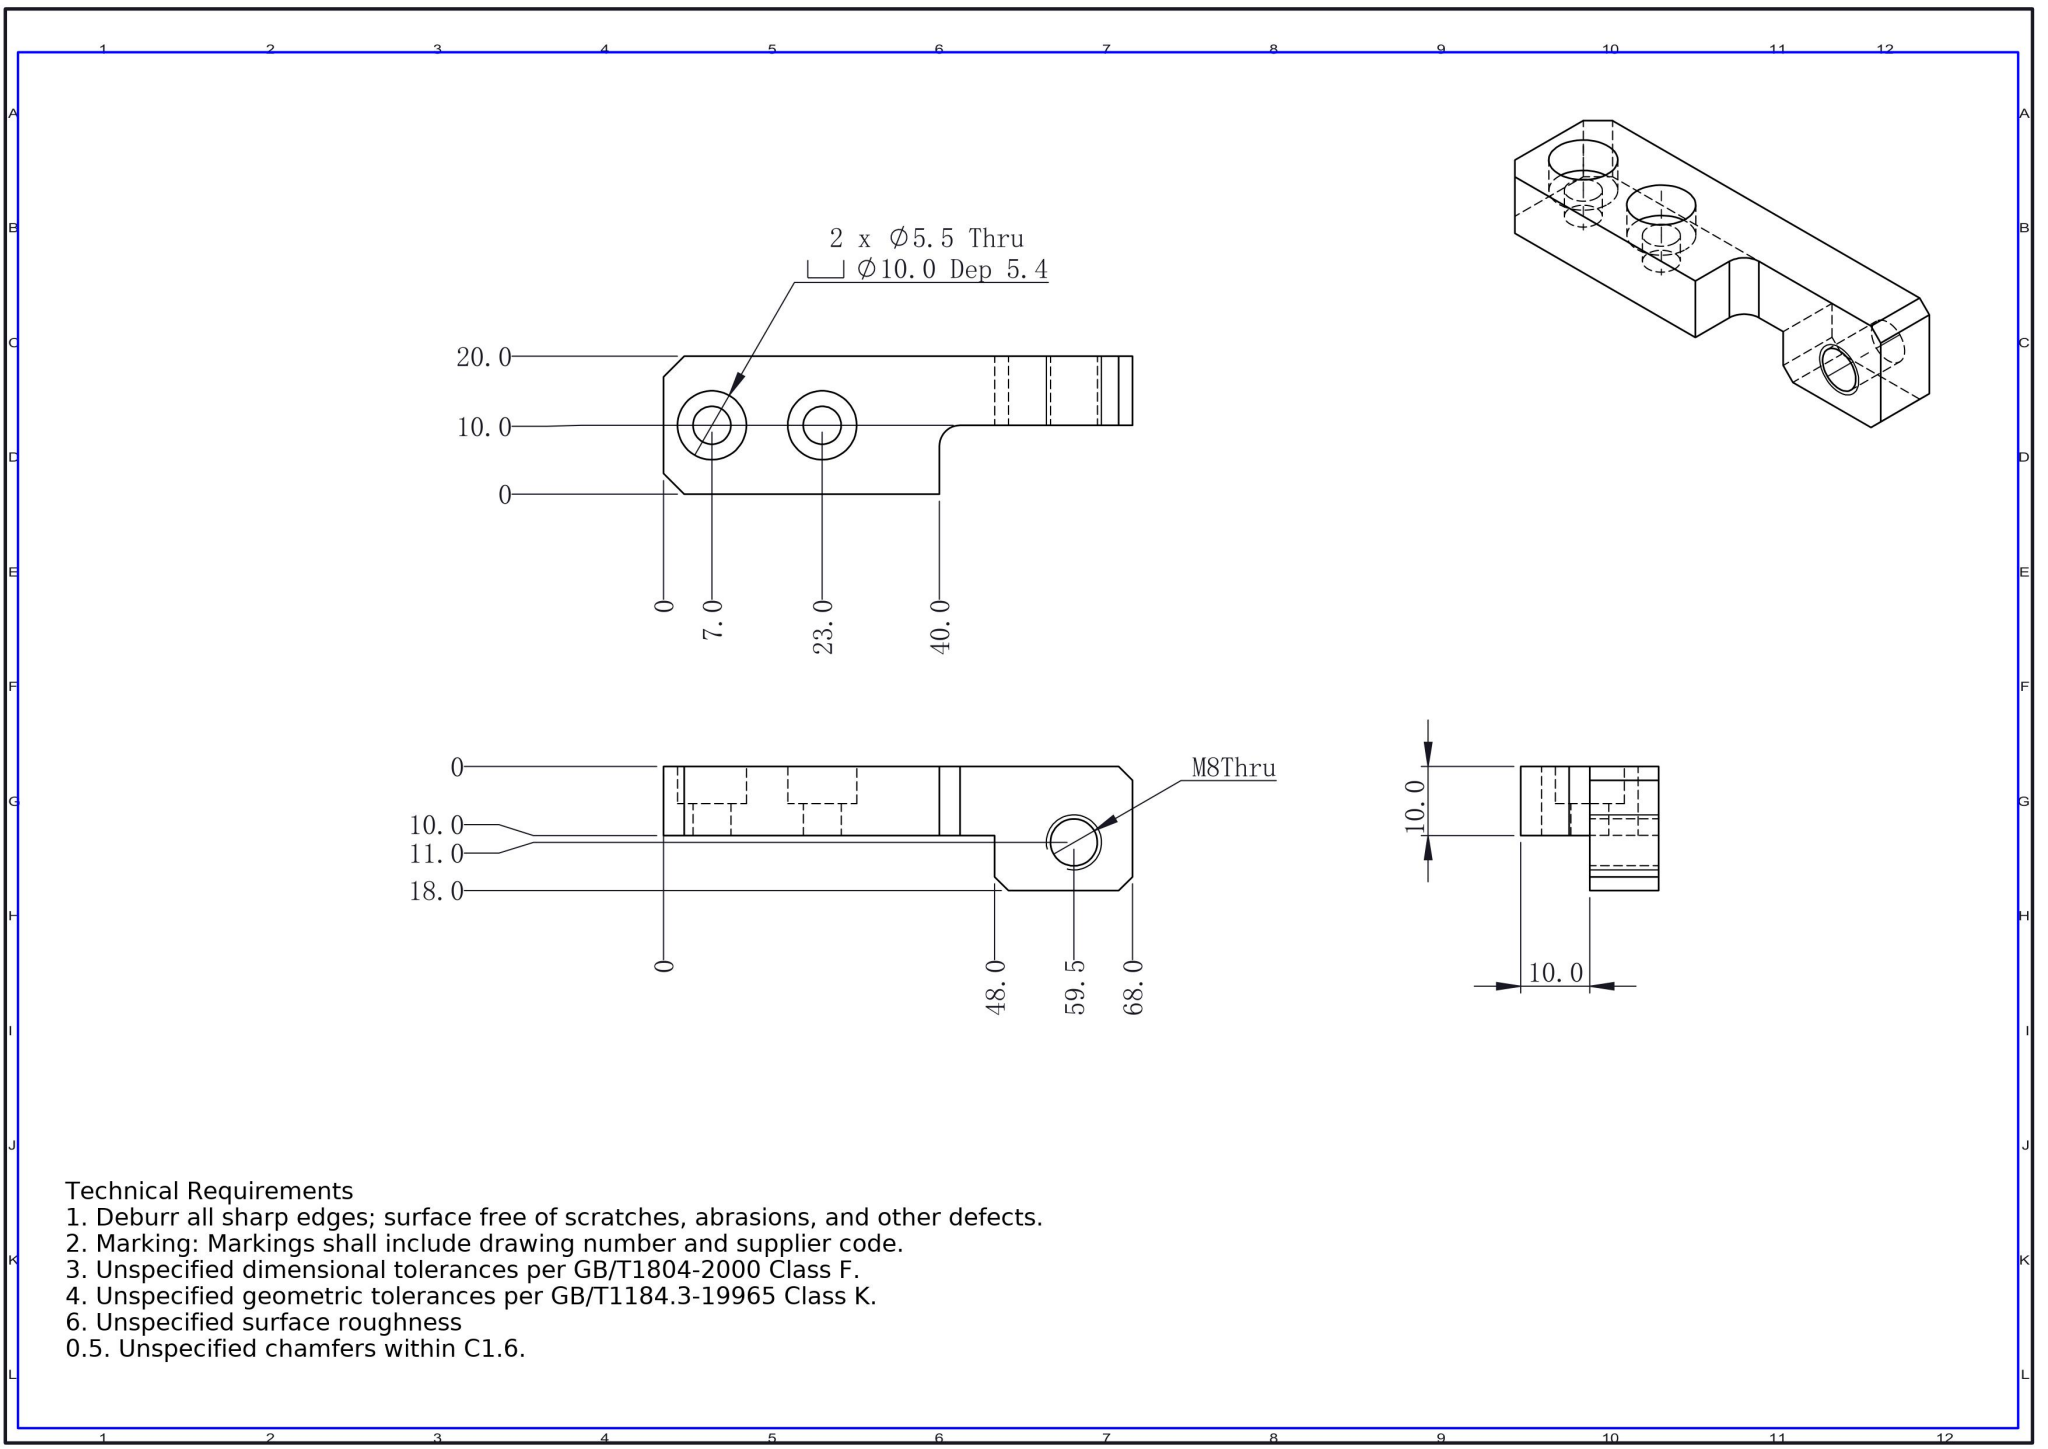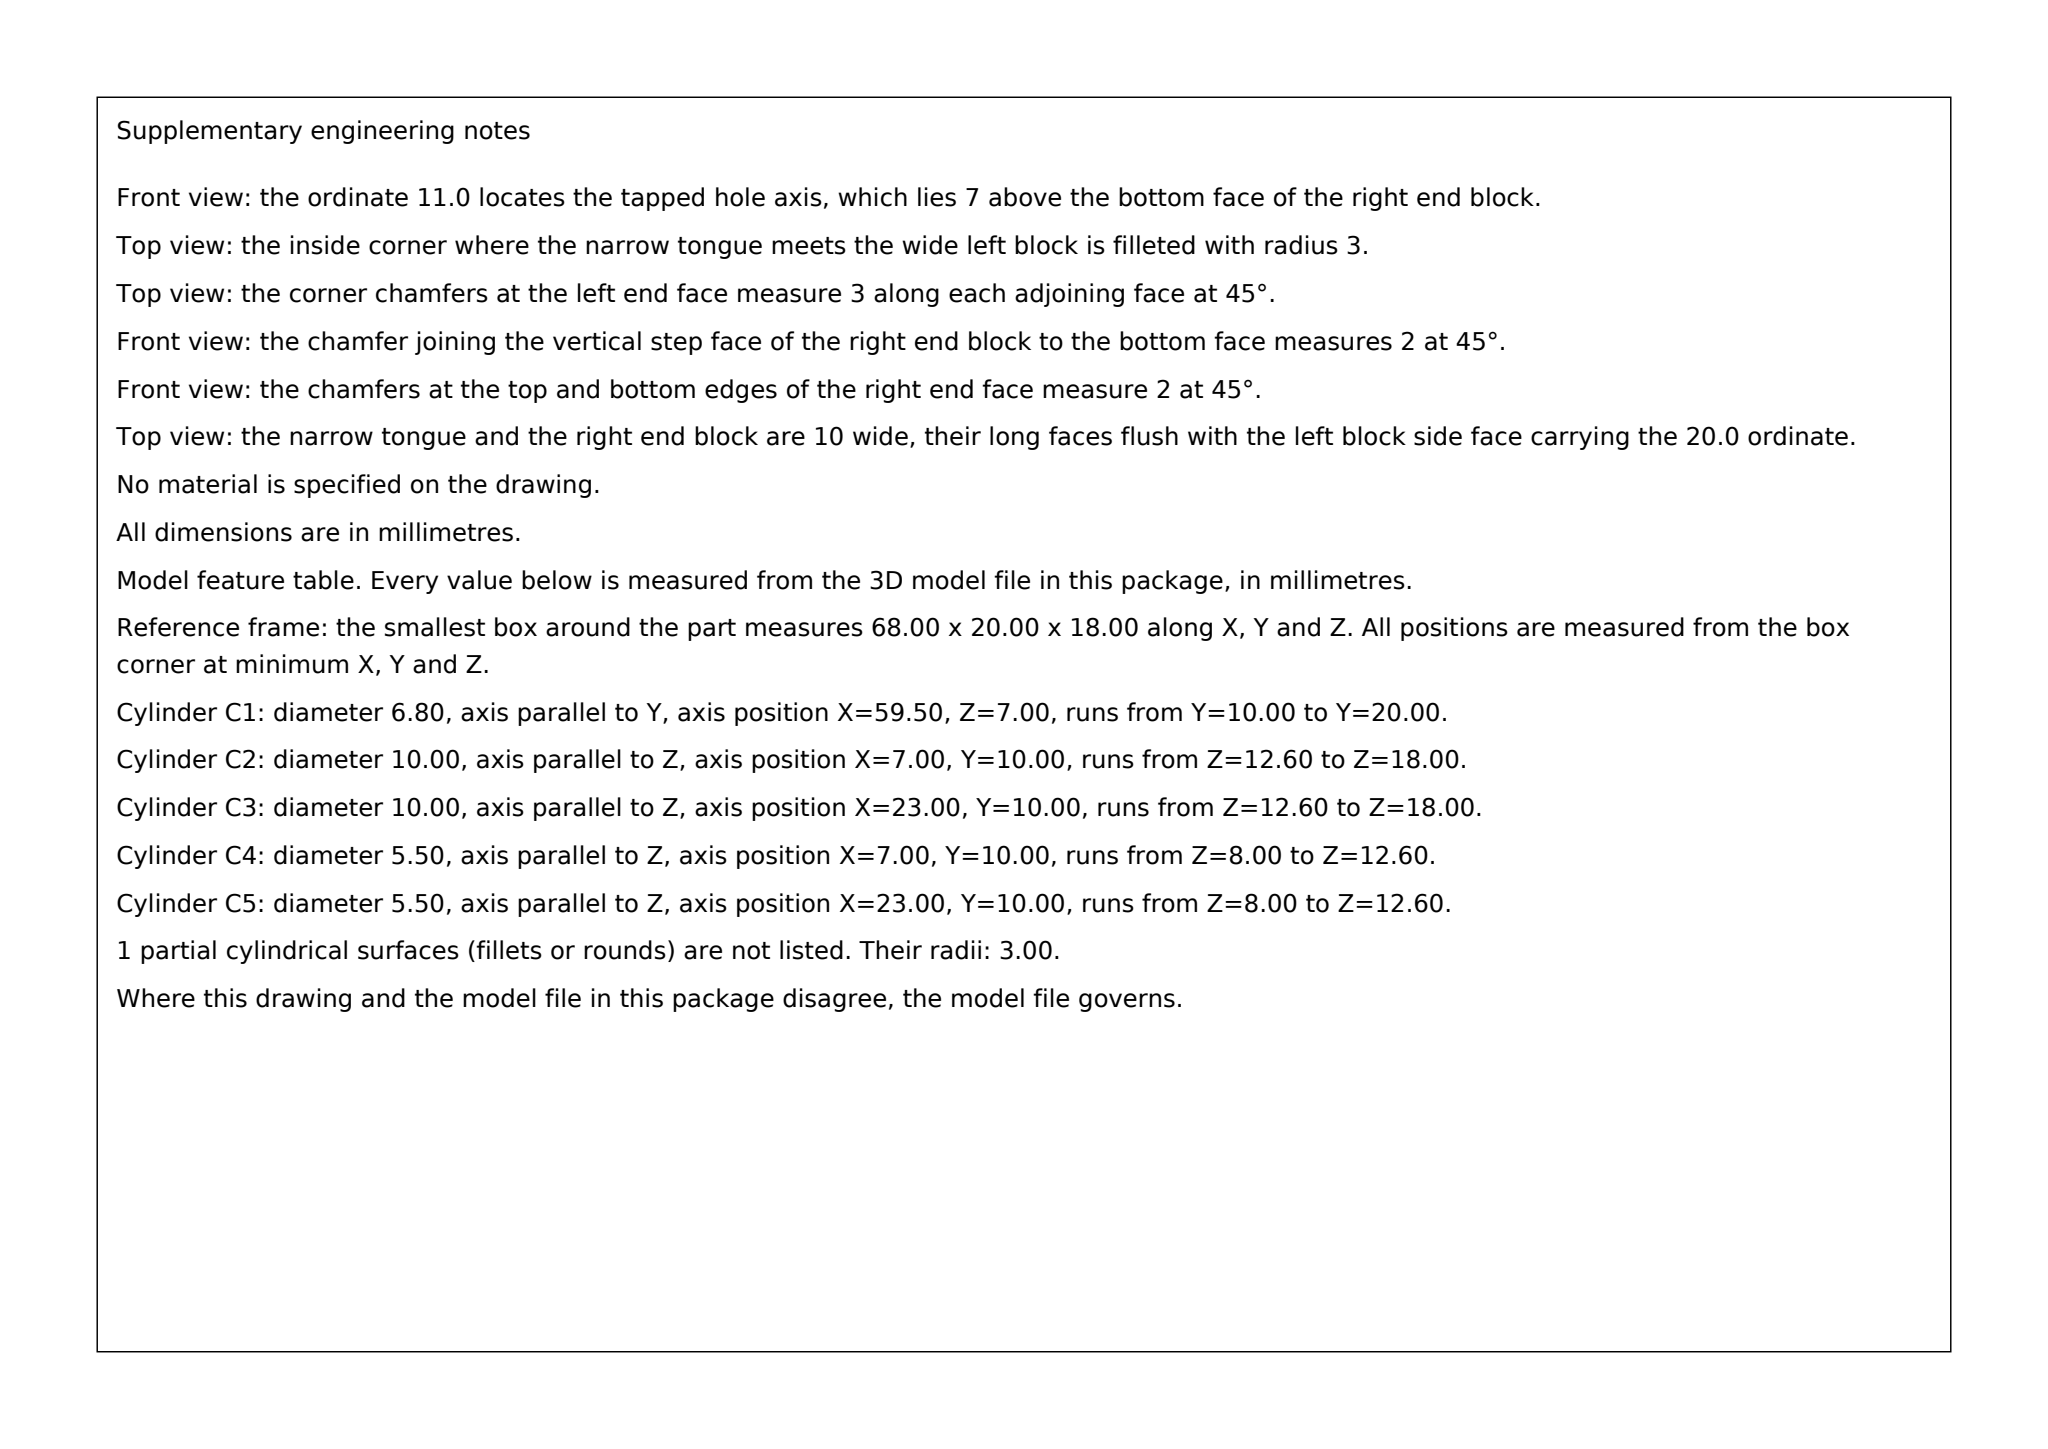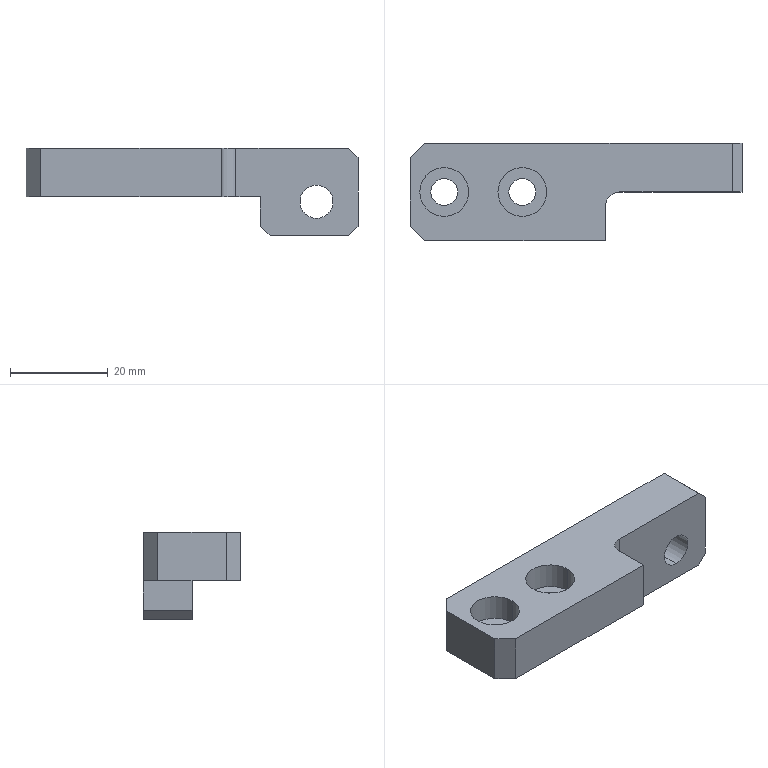Part | SolidWorks | mm | 1 solid | 28 faces | box 68 x 20 x 18 mm | volume 10839 mm3 | plane 17 | cylinder 11 | commonest cylinder face diameters 10 x4 5.5 x4 6.8 x2 6 x1
Drawing notes:
Ø6.0 DP 10.0 FROM TOP FACE; 43.0 FROM LEFT END, 7.0 FROM FRONT EDGE | from the solid: cylinder [6.0,'z',[43.0,7.0,null],10.0]; bbox 68x20x18; z-plane at 8.0 = hole bottom from top face z=18
build123d program:
from build123d import *

# Parameters (mm, degrees)
BOSS_EXTRUDE1_DEPTH                             = 18
M5_HEX_SOCKET_HEAD_CAP_SCREW_CBORE1_D           = 5.5
M5_HEX_SOCKET_HEAD_CAP_SCREW_CBORE1_CBORE_D     = 10
M5_HEX_SOCKET_HEAD_CAP_SCREW_CBORE1_CBORE_DEPTH = 5.4
CHAMFER1_SIZE                                   = 3
FILLET1_R                                       = 3
SKETCH6_W                                       = 48
SKETCH6_H                                       = 8
CUT_EXTRUDE1_DEPTH                              = 74.13
CHAMFER2_SIZE                                   = 2
M8_TAPPED_HOLE1_D                               = 6.8


with BuildPart() as part:
    # Sketch1 → Boss-Extrude1 (new body)
    with BuildSketch(Plane.XY):
        Polygon((0, 0), (68, 0), (68, -10), (40, -10), (40, -20), (0, -20), align=None)
    extrude(amount=BOSS_EXTRUDE1_DEPTH)

    # M5 Hex Socket Head Cap Screw CBORE1 (through all)
    with Locations(Plane.XY.offset(18)):
        with Locations((7, -10), (23, -10)):
            CounterBoreHole(M5_HEX_SOCKET_HEAD_CAP_SCREW_CBORE1_D / 2, M5_HEX_SOCKET_HEAD_CAP_SCREW_CBORE1_CBORE_D / 2, M5_HEX_SOCKET_HEAD_CAP_SCREW_CBORE1_CBORE_DEPTH)

    # Chamfer1
    chamfer1_edges = [part.edges().sort_by_distance(p)[0] for p in [
        (0, 0, 9),
        (0, -20, 9),
    ]]
    chamfer(chamfer1_edges, length=CHAMFER1_SIZE)

    # Fillet1
    fillet1_edges = [part.edges().sort_by_distance(p)[0] for p in [
        (40, -10, 9),
    ]]
    fillet(fillet1_edges, radius=FILLET1_R)

    # Sketch6 → Cut-Extrude1 (cut, through all)
    with BuildSketch(Plane.XZ.offset(20)):
        with Locations((24, 4)):
            Rectangle(SKETCH6_W, SKETCH6_H)
    extrude(amount=-CUT_EXTRUDE1_DEPTH, mode=Mode.SUBTRACT)

    # Chamfer2
    chamfer2_edges = [part.edges().sort_by_distance(p)[0] for p in [
        (68, -5, 18),
        (48, -5, 0),
        (68, -5, 0),
    ]]
    chamfer(chamfer2_edges, length=CHAMFER2_SIZE)

    # M8 Tapped Hole1 (through all)
    with Locations(Plane(origin=(0, -10, 0), x_dir=(-1, 0, 0), z_dir=(0, -1, 0))):
        with Locations((-59.5, -7)):
            Hole(M8_TAPPED_HOLE1_D / 2)


solid = part.part
STEP:
#1=CARTESIAN_POINT('',(59.5,0.,10.4));
#2=VERTEX_POINT('',#1);
#3=CARTESIAN_POINT('',(59.5,0.,3.6));
#4=VERTEX_POINT('',#3);
#5=CARTESIAN_POINT('',(59.5,0.,7.));
#6=DIRECTION('',(0.,-1.,0.));
#7=DIRECTION('',(0.,0.,-1.));
#8=AXIS2_PLACEMENT_3D('',#5,#6,#7);
#9=CIRCLE('',#8,3.4);
#10=EDGE_CURVE('',#2,#4,#9,.T.);
#11=ORIENTED_EDGE('',*,*,#10,.F.);
#12=CARTESIAN_POINT('',(59.5,-10.,10.4));
#13=VERTEX_POINT('',#12);
#14=CARTESIAN_POINT('',(59.5,-10.,10.4));
#15=DIRECTION('',(0.,-1.,0.));
#16=VECTOR('',#15,1000.);
#17=LINE('',#14,#16);
#18=EDGE_CURVE('',#2,#13,#17,.T.);
#19=ORIENTED_EDGE('',*,*,#18,.T.);
#20=CARTESIAN_POINT('',(59.5,-10.,3.6));
#21=VERTEX_POINT('',#20);
#22=CARTESIAN_POINT('',(59.5,-10.,7.));
#23=DIRECTION('',(0.,-1.,0.));
#24=DIRECTION('',(0.,0.,-1.));
#25=AXIS2_PLACEMENT_3D('',#22,#23,#24);
#26=CIRCLE('',#25,3.4);
#27=EDGE_CURVE('',#13,#21,#26,.T.);
#28=ORIENTED_EDGE('',*,*,#27,.T.);
#29=CARTESIAN_POINT('',(59.5,-10.,3.6));
#30=DIRECTION('',(0.,-1.,0.));
#31=VECTOR('',#30,1000.);
#32=LINE('',#29,#31);
#33=EDGE_CURVE('',#4,#21,#32,.T.);
#34=ORIENTED_EDGE('',*,*,#33,.F.);
#35=EDGE_LOOP('',(#11,#19,#28,#34));
#36=FACE_OUTER_BOUND('',#35,.T.);
#37=CARTESIAN_POINT('',(59.5,-10.,7.));
#38=DIRECTION('',(0.,-1.,0.));
#39=DIRECTION('',(0.,0.,-1.));
#40=AXIS2_PLACEMENT_3D('',#37,#38,#39);
#41=CYLINDRICAL_SURFACE('',#40,3.4);
#42=ADVANCED_FACE('',(#36),#41,.F.);
#43=CARTESIAN_POINT('',(2.,-10.,12.6));
#44=VERTEX_POINT('',#43);
#45=CARTESIAN_POINT('',(12.,-10.,12.6));
#46=VERTEX_POINT('',#45);
#47=CARTESIAN_POINT('',(7.,-10.,12.6));
#48=DIRECTION('',(0.,0.,1.));
#49=DIRECTION('',(1.,0.,0.));
#50=AXIS2_PLACEMENT_3D('',#47,#48,#49);
#51=CIRCLE('',#50,5.);
#52=EDGE_CURVE('',#44,#46,#51,.T.);
#53=ORIENTED_EDGE('',*,*,#52,.F.);
#54=CARTESIAN_POINT('',(2.,-10.,18.));
#55=VERTEX_POINT('',#54);
#56=CARTESIAN_POINT('',(2.,-10.,18.));
#57=DIRECTION('',(0.,0.,1.));
#58=VECTOR('',#57,1000.);
#59=LINE('',#56,#58);
#60=EDGE_CURVE('',#44,#55,#59,.T.);
#61=ORIENTED_EDGE('',*,*,#60,.T.);
#62=CARTESIAN_POINT('',(12.,-10.,18.));
#63=VERTEX_POINT('',#62);
#64=CARTESIAN_POINT('',(7.,-10.,18.));
#65=DIRECTION('',(0.,0.,1.));
#66=DIRECTION('',(1.,0.,0.));
#67=AXIS2_PLACEMENT_3D('',#64,#65,#66);
#68=CIRCLE('',#67,5.);
#69=EDGE_CURVE('',#55,#63,#68,.T.);
#70=ORIENTED_EDGE('',*,*,#69,.T.);
#71=CARTESIAN_POINT('',(12.,-10.,18.));
#72=DIRECTION('',(0.,0.,1.));
#73=VECTOR('',#72,1000.);
#74=LINE('',#71,#73);
#75=EDGE_CURVE('',#46,#63,#74,.T.);
#76=ORIENTED_EDGE('',*,*,#75,.F.);
#77=EDGE_LOOP('',(#53,#61,#70,#76));
#78=FACE_OUTER_BOUND('',#77,.T.);
#79=CARTESIAN_POINT('',(7.,-10.,18.));
#80=DIRECTION('',(0.,0.,1.));
#81=DIRECTION('',(1.,0.,0.));
#82=AXIS2_PLACEMENT_3D('',#79,#80,#81);
#83=CYLINDRICAL_SURFACE('',#82,5.);
#84=ADVANCED_FACE('',(#78),#83,.F.);
#85=CARTESIAN_POINT('',(9.75,-10.,8.));
#86=VERTEX_POINT('',#85);
#87=CARTESIAN_POINT('',(4.25,-10.,8.));
#88=VERTEX_POINT('',#87);
#89=CARTESIAN_POINT('',(7.,-10.,8.));
#90=DIRECTION('',(0.,0.,-1.));
#91=DIRECTION('',(1.,0.,0.));
#92=AXIS2_PLACEMENT_3D('',#89,#90,#91);
#93=CIRCLE('',#92,2.75);
#94=EDGE_CURVE('',#86,#88,#93,.T.);
#95=ORIENTED_EDGE('',*,*,#94,.T.);
#96=CARTESIAN_POINT('',(4.25,-10.,12.6));
#97=VERTEX_POINT('',#96);
#98=CARTESIAN_POINT('',(4.25,-10.,18.));
#99=DIRECTION('',(0.,0.,1.));
#100=VECTOR('',#99,1000.);
#101=LINE('',#98,#100);
#102=EDGE_CURVE('',#88,#97,#101,.T.);
#103=ORIENTED_EDGE('',*,*,#102,.T.);
#104=CARTESIAN_POINT('',(9.75,-10.,12.6));
#105=VERTEX_POINT('',#104);
#106=CARTESIAN_POINT('',(7.,-10.,12.6));
#107=DIRECTION('',(0.,0.,1.));
#108=DIRECTION('',(1.,0.,0.));
#109=AXIS2_PLACEMENT_3D('',#106,#107,#108);
#110=CIRCLE('',#109,2.75);
#111=EDGE_CURVE('',#97,#105,#110,.T.);
#112=ORIENTED_EDGE('',*,*,#111,.T.);
#113=CARTESIAN_POINT('',(9.75,-10.,18.));
#114=DIRECTION('',(0.,0.,1.));
#115=VECTOR('',#114,1000.);
#116=LINE('',#113,#115);
#117=EDGE_CURVE('',#86,#105,#116,.T.);
#118=ORIENTED_EDGE('',*,*,#117,.F.);
#119=EDGE_LOOP('',(#95,#103,#112,#118));
#120=FACE_OUTER_BOUND('',#119,.T.);
#121=CARTESIAN_POINT('',(7.,-10.,18.));
#122=DIRECTION('',(0.,0.,1.));
#123=DIRECTION('',(1.,0.,0.));
#124=AXIS2_PLACEMENT_3D('',#121,#122,#123);
#125=CYLINDRICAL_SURFACE('',#124,2.75);
#126=ADVANCED_FACE('',(#120),#125,.F.);
#127=CARTESIAN_POINT('',(18.,-10.,12.6));
#128=VERTEX_POINT('',#127);
#129=CARTESIAN_POINT('',(28.,-10.,12.6));
#130=VERTEX_POINT('',#129);
#131=CARTESIAN_POINT('',(23.,-10.,12.6));
#132=DIRECTION('',(0.,0.,1.));
#133=DIRECTION('',(1.,0.,0.));
#134=AXIS2_PLACEMENT_3D('',#131,#132,#133);
#135=CIRCLE('',#134,5.);
#136=EDGE_CURVE('',#128,#130,#135,.T.);
#137=ORIENTED_EDGE('',*,*,#136,.F.);
#138=CARTESIAN_POINT('',(18.,-10.,18.));
#139=VERTEX_POINT('',#138);
#140=CARTESIAN_POINT('',(18.,-10.,18.));
#141=DIRECTION('',(0.,0.,1.));
#142=VECTOR('',#141,1000.);
#143=LINE('',#140,#142);
#144=EDGE_CURVE('',#128,#139,#143,.T.);
#145=ORIENTED_EDGE('',*,*,#144,.T.);
#146=CARTESIAN_POINT('',(28.,-10.,18.));
#147=VERTEX_POINT('',#146);
#148=CARTESIAN_POINT('',(23.,-10.,18.));
#149=DIRECTION('',(0.,0.,1.));
#150=DIRECTION('',(1.,0.,0.));
#151=AXIS2_PLACEMENT_3D('',#148,#149,#150);
#152=CIRCLE('',#151,5.);
#153=EDGE_CURVE('',#139,#147,#152,.T.);
#154=ORIENTED_EDGE('',*,*,#153,.T.);
#155=CARTESIAN_POINT('',(28.,-10.,18.));
#156=DIRECTION('',(0.,0.,1.));
#157=VECTOR('',#156,1000.);
#158=LINE('',#155,#157);
#159=EDGE_CURVE('',#130,#147,#158,.T.);
#160=ORIENTED_EDGE('',*,*,#159,.F.);
#161=EDGE_LOOP('',(#137,#145,#154,#160));
#162=FACE_OUTER_BOUND('',#161,.T.);
#163=CARTESIAN_POINT('',(23.,-10.,18.));
#164=DIRECTION('',(0.,0.,1.));
#165=DIRECTION('',(1.,0.,0.));
#166=AXIS2_PLACEMENT_3D('',#163,#164,#165);
#167=CYLINDRICAL_SURFACE('',#166,5.);
#168=ADVANCED_FACE('',(#162),#167,.F.);
#169=CARTESIAN_POINT('',(25.75,-10.,8.));
#170=VERTEX_POINT('',#169);
#171=CARTESIAN_POINT('',(20.25,-10.,8.));
#172=VERTEX_POINT('',#171);
#173=CARTESIAN_POINT('',(23.,-10.,8.));
#174=DIRECTION('',(0.,0.,-1.));
#175=DIRECTION('',(1.,0.,0.));
#176=AXIS2_PLACEMENT_3D('',#173,#174,#175);
#177=CIRCLE('',#176,2.75);
#178=EDGE_CURVE('',#170,#172,#177,.T.);
#179=ORIENTED_EDGE('',*,*,#178,.T.);
#180=CARTESIAN_POINT('',(20.25,-10.,12.6));
#181=VERTEX_POINT('',#180);
#182=CARTESIAN_POINT('',(20.25,-10.,18.));
#183=DIRECTION('',(0.,0.,1.));
#184=VECTOR('',#183,1000.);
#185=LINE('',#182,#184);
#186=EDGE_CURVE('',#172,#181,#185,.T.);
#187=ORIENTED_EDGE('',*,*,#186,.T.);
#188=CARTESIAN_POINT('',(25.75,-10.,12.6));
#189=VERTEX_POINT('',#188);
#190=CARTESIAN_POINT('',(23.,-10.,12.6));
#191=DIRECTION('',(0.,0.,1.));
#192=DIRECTION('',(1.,0.,0.));
#193=AXIS2_PLACEMENT_3D('',#190,#191,#192);
#194=CIRCLE('',#193,2.75);
#195=EDGE_CURVE('',#181,#189,#194,.T.);
#196=ORIENTED_EDGE('',*,*,#195,.T.);
#197=CARTESIAN_POINT('',(25.75,-10.,18.));
#198=DIRECTION('',(0.,0.,1.));
#199=VECTOR('',#198,1000.);
#200=LINE('',#197,#199);
#201=EDGE_CURVE('',#170,#189,#200,.T.);
#202=ORIENTED_EDGE('',*,*,#201,.F.);
#203=EDGE_LOOP('',(#179,#187,#196,#202));
#204=FACE_OUTER_BOUND('',#203,.T.);
#205=CARTESIAN_POINT('',(23.,-10.,18.));
#206=DIRECTION('',(0.,0.,1.));
#207=DIRECTION('',(1.,0.,0.));
#208=AXIS2_PLACEMENT_3D('',#205,#206,#207);
#209=CYLINDRICAL_SURFACE('',#208,2.75);
#210=ADVANCED_FACE('',(#204),#209,.F.);
#211=CARTESIAN_POINT('',(0.,-3.,18.));
#212=VERTEX_POINT('',#211);
#213=CARTESIAN_POINT('',(0.,-3.,8.));
#214=VERTEX_POINT('',#213);
#215=CARTESIAN_POINT('',(0.,-3.,18.));
#216=DIRECTION('',(0.,0.,-1.));
#217=VECTOR('',#216,1000.);
#218=LINE('',#215,#217);
#219=EDGE_CURVE('',#212,#214,#218,.T.);
#220=ORIENTED_EDGE('',*,*,#219,.T.);
#221=CARTESIAN_POINT('',(-0.,-17.,8.));
#222=VERTEX_POINT('',#221);
#223=CARTESIAN_POINT('',(0.,0.,8.));
#224=DIRECTION('',(0.,-1.,0.));
#225=VECTOR('',#224,1000.);
#226=LINE('',#223,#225);
#227=EDGE_CURVE('',#214,#222,#226,.T.);
#228=ORIENTED_EDGE('',*,*,#227,.T.);
#229=CARTESIAN_POINT('',(0.,-17.,18.));
#230=VERTEX_POINT('',#229);
#231=CARTESIAN_POINT('',(0.,-17.,18.));
#232=DIRECTION('',(0.,0.,1.));
#233=VECTOR('',#232,1000.);
#234=LINE('',#231,#233);
#235=EDGE_CURVE('',#222,#230,#234,.T.);
#236=ORIENTED_EDGE('',*,*,#235,.T.);
#237=CARTESIAN_POINT('',(0.,0.,18.));
#238=DIRECTION('',(0.,-1.,0.));
#239=VECTOR('',#238,1000.);
#240=LINE('',#237,#239);
#241=EDGE_CURVE('',#212,#230,#240,.T.);
#242=ORIENTED_EDGE('',*,*,#241,.F.);
#243=EDGE_LOOP('',(#220,#228,#236,#242));
#244=FACE_OUTER_BOUND('',#243,.T.);
#245=CARTESIAN_POINT('',(0.,0.,18.));
#246=DIRECTION('',(1.,0.,0.));
#247=DIRECTION('',(0.,0.,-1.));
#248=AXIS2_PLACEMENT_3D('',#245,#246,#247);
#249=PLANE('',#248);
#250=ADVANCED_FACE('',(#244),#249,.F.);
#251=CARTESIAN_POINT('',(3.,-20.,18.));
#252=VERTEX_POINT('',#251);
#253=CARTESIAN_POINT('',(3.,-20.,8.));
#254=VERTEX_POINT('',#253);
#255=CARTESIAN_POINT('',(3.,-20.,18.));
#256=DIRECTION('',(0.,0.,-1.));
#257=VECTOR('',#256,1000.);
#258=LINE('',#255,#257);
#259=EDGE_CURVE('',#252,#254,#258,.T.);
#260=ORIENTED_EDGE('',*,*,#259,.T.);
#261=CARTESIAN_POINT('',(40.,-20.,8.));
#262=VERTEX_POINT('',#261);
#263=CARTESIAN_POINT('',(0.,-20.,8.));
#264=DIRECTION('',(-1.,0.,0.));
#265=VECTOR('',#264,1000.);
#266=LINE('',#263,#265);
#267=EDGE_CURVE('',#262,#254,#266,.T.);
#268=ORIENTED_EDGE('',*,*,#267,.F.);
#269=CARTESIAN_POINT('',(40.,-20.,18.));
#270=VERTEX_POINT('',#269);
#271=CARTESIAN_POINT('',(40.,-20.,18.));
#272=DIRECTION('',(0.,0.,-1.));
#273=VECTOR('',#272,1000.);
#274=LINE('',#271,#273);
#275=EDGE_CURVE('',#270,#262,#274,.T.);
#276=ORIENTED_EDGE('',*,*,#275,.F.);
#277=CARTESIAN_POINT('',(0.,-20.,18.));
#278=DIRECTION('',(1.,0.,0.));
#279=VECTOR('',#278,1000.);
#280=LINE('',#277,#279);
#281=EDGE_CURVE('',#252,#270,#280,.T.);
#282=ORIENTED_EDGE('',*,*,#281,.F.);
#283=EDGE_LOOP('',(#260,#268,#276,#282));
#284=FACE_OUTER_BOUND('',#283,.T.);
#285=CARTESIAN_POINT('',(0.,-20.,18.));
#286=DIRECTION('',(0.,1.,0.));
#287=DIRECTION('',(0.,0.,1.));
#288=AXIS2_PLACEMENT_3D('',#285,#286,#287);
#289=PLANE('',#288);
#290=ADVANCED_FACE('',(#284),#289,.F.);
#291=ORIENTED_EDGE('',*,*,#275,.T.);
#292=CARTESIAN_POINT('',(40.,-13.,8.));
#293=VERTEX_POINT('',#292);
#294=CARTESIAN_POINT('',(40.,-20.,8.));
#295=DIRECTION('',(0.,1.,0.));
#296=VECTOR('',#295,1000.);
#297=LINE('',#294,#296);
#298=EDGE_CURVE('',#262,#293,#297,.T.);
#299=ORIENTED_EDGE('',*,*,#298,.T.);
#300=CARTESIAN_POINT('',(40.,-13.,18.));
#301=VERTEX_POINT('',#300);
#302=CARTESIAN_POINT('',(40.,-13.,18.));
#303=DIRECTION('',(0.,0.,1.));
#304=VECTOR('',#303,1000.);
#305=LINE('',#302,#304);
#306=EDGE_CURVE('',#293,#301,#305,.T.);
#307=ORIENTED_EDGE('',*,*,#306,.T.);
#308=CARTESIAN_POINT('',(40.,-20.,18.));
#309=DIRECTION('',(0.,1.,0.));
#310=VECTOR('',#309,1000.);
#311=LINE('',#308,#310);
#312=EDGE_CURVE('',#270,#301,#311,.T.);
#313=ORIENTED_EDGE('',*,*,#312,.F.);
#314=EDGE_LOOP('',(#291,#299,#307,#313));
#315=FACE_OUTER_BOUND('',#314,.T.);
#316=CARTESIAN_POINT('',(40.,-20.,18.));
#317=DIRECTION('',(-1.,0.,0.));
#318=DIRECTION('',(0.,0.,1.));
#319=AXIS2_PLACEMENT_3D('',#316,#317,#318);
#320=PLANE('',#319);
#321=ADVANCED_FACE('',(#315),#320,.F.);
#322=CARTESIAN_POINT('',(59.5,-10.,7.));
#323=DIRECTION('',(0.,-1.,0.));
#324=DIRECTION('',(0.,0.,-1.));
#325=AXIS2_PLACEMENT_3D('',#322,#323,#324);
#326=CIRCLE('',#325,3.4);
#327=EDGE_CURVE('',#21,#13,#326,.T.);
#328=ORIENTED_EDGE('',*,*,#327,.F.);
#329=ORIENTED_EDGE('',*,*,#27,.F.);
#330=EDGE_LOOP('',(#328,#329));
#331=FACE_BOUND('',#330,.T.);
#332=CARTESIAN_POINT('',(48.,-10.,8.));
#333=VERTEX_POINT('',#332);
#334=CARTESIAN_POINT('',(48.,-10.,2.));
#335=VERTEX_POINT('',#334);
#336=CARTESIAN_POINT('',(48.,-10.,18.));
#337=DIRECTION('',(0.,0.,-1.));
#338=VECTOR('',#337,1000.);
#339=LINE('',#336,#338);
#340=EDGE_CURVE('',#333,#335,#339,.T.);
#341=ORIENTED_EDGE('',*,*,#340,.T.);
#342=CARTESIAN_POINT('',(50.,-10.,0.));
#343=VERTEX_POINT('',#342);
#344=CARTESIAN_POINT('',(48.,-10.,2.));
#345=DIRECTION('',(0.7071,0.,-0.7071));
#346=VECTOR('',#345,1000.);
#347=LINE('',#344,#346);
#348=EDGE_CURVE('',#335,#343,#347,.T.);
#349=ORIENTED_EDGE('',*,*,#348,.T.);
#350=CARTESIAN_POINT('',(66.,-10.,0.));
#351=VERTEX_POINT('',#350);
#352=CARTESIAN_POINT('',(68.,-10.,0.));
#353=DIRECTION('',(1.,0.,0.));
#354=VECTOR('',#353,1000.);
#355=LINE('',#352,#354);
#356=EDGE_CURVE('',#343,#351,#355,.T.);
#357=ORIENTED_EDGE('',*,*,#356,.T.);
#358=CARTESIAN_POINT('',(68.,-10.,2.));
#359=VERTEX_POINT('',#358);
#360=CARTESIAN_POINT('',(68.,-10.,2.));
#361=DIRECTION('',(0.7071,0.,0.7071));
#362=VECTOR('',#361,1000.);
#363=LINE('',#360,#362);
#364=EDGE_CURVE('',#351,#359,#363,.T.);
#365=ORIENTED_EDGE('',*,*,#364,.T.);
#366=CARTESIAN_POINT('',(68.,-10.,16.));
#367=VERTEX_POINT('',#366);
#368=CARTESIAN_POINT('',(68.,-10.,18.));
#369=DIRECTION('',(0.,0.,-1.));
#370=VECTOR('',#369,1000.);
#371=LINE('',#368,#370);
#372=EDGE_CURVE('',#367,#359,#371,.T.);
#373=ORIENTED_EDGE('',*,*,#372,.F.);
#374=CARTESIAN_POINT('',(66.,-10.,18.));
#375=VERTEX_POINT('',#374);
#376=CARTESIAN_POINT('',(66.,-10.,18.));
#377=DIRECTION('',(-0.7071,-0.,0.7071));
#378=VECTOR('',#377,1000.);
#379=LINE('',#376,#378);
#380=EDGE_CURVE('',#367,#375,#379,.T.);
#381=ORIENTED_EDGE('',*,*,#380,.T.);
#382=CARTESIAN_POINT('',(43.,-10.,18.));
#383=VERTEX_POINT('',#382);
#384=CARTESIAN_POINT('',(68.,-10.,18.));
#385=DIRECTION('',(1.,0.,0.));
#386=VECTOR('',#385,1000.);
#387=LINE('',#384,#386);
#388=EDGE_CURVE('',#383,#375,#387,.T.);
#389=ORIENTED_EDGE('',*,*,#388,.F.);
#390=CARTESIAN_POINT('',(43.,-10.,8.));
#391=VERTEX_POINT('',#390);
#392=CARTESIAN_POINT('',(43.,-10.,0.));
#393=DIRECTION('',(0.,0.,-1.));
#394=VECTOR('',#393,1000.);
#395=LINE('',#392,#394);
#396=EDGE_CURVE('',#383,#391,#395,.T.);
#397=ORIENTED_EDGE('',*,*,#396,.T.);
#398=CARTESIAN_POINT('',(68.,-10.,8.));
#399=DIRECTION('',(1.,0.,0.));
#400=VECTOR('',#399,1000.);
#401=LINE('',#398,#400);
#402=EDGE_CURVE('',#391,#333,#401,.T.);
#403=ORIENTED_EDGE('',*,*,#402,.T.);
#404=EDGE_LOOP('',(#341,#349,#357,#365,#373,#381,#389,#397,#403));
#405=FACE_OUTER_BOUND('',#404,.T.);
#406=CARTESIAN_POINT('',(68.,-10.,18.));
#407=DIRECTION('',(-0.,1.,0.));
#408=DIRECTION('',(-1.,-0.,0.));
#409=AXIS2_PLACEMENT_3D('',#406,#407,#408);
#410=PLANE('',#409);
#411=ADVANCED_FACE('',(#331,#405),#410,.F.);
#412=ORIENTED_EDGE('',*,*,#372,.T.);
#413=CARTESIAN_POINT('',(68.,0.,2.));
#414=VERTEX_POINT('',#413);
#415=CARTESIAN_POINT('',(68.,0.,2.));
#416=DIRECTION('',(0.,1.,0.));
#417=VECTOR('',#416,1000.);
#418=LINE('',#415,#417);
#419=EDGE_CURVE('',#359,#414,#418,.T.);
#420=ORIENTED_EDGE('',*,*,#419,.T.);
#421=CARTESIAN_POINT('',(68.,0.,16.));
#422=VERTEX_POINT('',#421);
#423=CARTESIAN_POINT('',(68.,0.,18.));
#424=DIRECTION('',(0.,0.,-1.));
#425=VECTOR('',#424,1000.);
#426=LINE('',#423,#425);
#427=EDGE_CURVE('',#422,#414,#426,.T.);
#428=ORIENTED_EDGE('',*,*,#427,.F.);
#429=CARTESIAN_POINT('',(68.,-10.,16.));
#430=DIRECTION('',(0.,-1.,0.));
#431=VECTOR('',#430,1000.);
#432=LINE('',#429,#431);
#433=EDGE_CURVE('',#422,#367,#432,.T.);
#434=ORIENTED_EDGE('',*,*,#433,.T.);
#435=EDGE_LOOP('',(#412,#420,#428,#434));
#436=FACE_OUTER_BOUND('',#435,.T.);
#437=CARTESIAN_POINT('',(68.,0.,18.));
#438=DIRECTION('',(-1.,0.,0.));
#439=DIRECTION('',(0.,0.,1.));
#440=AXIS2_PLACEMENT_3D('',#437,#438,#439);
#441=PLANE('',#440);
#442=ADVANCED_FACE('',(#436),#441,.F.);
#443=CARTESIAN_POINT('',(59.5,0.,7.));
#444=DIRECTION('',(0.,-1.,0.));
#445=DIRECTION('',(0.,0.,-1.));
#446=AXIS2_PLACEMENT_3D('',#443,#444,#445);
#447=CIRCLE('',#446,3.4);
#448=EDGE_CURVE('',#4,#2,#447,.T.);
#449=ORIENTED_EDGE('',*,*,#448,.T.);
#450=ORIENTED_EDGE('',*,*,#10,.T.);
#451=EDGE_LOOP('',(#449,#450));
#452=FACE_BOUND('',#451,.T.);
#453=CARTESIAN_POINT('',(66.,0.,0.));
#454=VERTEX_POINT('',#453);
#455=CARTESIAN_POINT('',(50.,0.,0.));
#456=VERTEX_POINT('',#455);
#457=CARTESIAN_POINT('',(0.,0.,0.));
#458=DIRECTION('',(-1.,0.,0.));
#459=VECTOR('',#458,1000.);
#460=LINE('',#457,#459);
#461=EDGE_CURVE('',#454,#456,#460,.T.);
#462=ORIENTED_EDGE('',*,*,#461,.T.);
#463=CARTESIAN_POINT('',(48.,0.,2.));
#464=VERTEX_POINT('',#463);
#465=CARTESIAN_POINT('',(48.,0.,2.));
#466=DIRECTION('',(-0.7071,0.,0.7071));
#467=VECTOR('',#466,1000.);
#468=LINE('',#465,#467);
#469=EDGE_CURVE('',#456,#464,#468,.T.);
#470=ORIENTED_EDGE('',*,*,#469,.T.);
#471=CARTESIAN_POINT('',(48.,0.,8.));
#472=VERTEX_POINT('',#471);
#473=CARTESIAN_POINT('',(48.,0.,0.));
#474=DIRECTION('',(0.,0.,1.));
#475=VECTOR('',#474,1000.);
#476=LINE('',#473,#475);
#477=EDGE_CURVE('',#464,#472,#476,.T.);
#478=ORIENTED_EDGE('',*,*,#477,.T.);
#479=CARTESIAN_POINT('',(3.,0.,8.));
#480=VERTEX_POINT('',#479);
#481=CARTESIAN_POINT('',(0.,0.,8.));
#482=DIRECTION('',(-1.,0.,0.));
#483=VECTOR('',#482,1000.);
#484=LINE('',#481,#483);
#485=EDGE_CURVE('',#472,#480,#484,.T.);
#486=ORIENTED_EDGE('',*,*,#485,.T.);
#487=CARTESIAN_POINT('',(3.,0.,18.));
#488=VERTEX_POINT('',#487);
#489=CARTESIAN_POINT('',(3.,0.,18.));
#490=DIRECTION('',(0.,0.,1.));
#491=VECTOR('',#490,1000.);
#492=LINE('',#489,#491);
#493=EDGE_CURVE('',#480,#488,#492,.T.);
#494=ORIENTED_EDGE('',*,*,#493,.T.);
#495=CARTESIAN_POINT('',(66.,0.,18.));
#496=VERTEX_POINT('',#495);
#497=CARTESIAN_POINT('',(0.,0.,18.));
#498=DIRECTION('',(-1.,0.,0.));
#499=VECTOR('',#498,1000.);
#500=LINE('',#497,#499);
#501=EDGE_CURVE('',#496,#488,#500,.T.);
#502=ORIENTED_EDGE('',*,*,#501,.F.);
#503=CARTESIAN_POINT('',(66.,0.,18.));
#504=DIRECTION('',(0.7071,0.,-0.7071));
#505=VECTOR('',#504,1000.);
#506=LINE('',#503,#505);
#507=EDGE_CURVE('',#496,#422,#506,.T.);
#508=ORIENTED_EDGE('',*,*,#507,.T.);
#509=ORIENTED_EDGE('',*,*,#427,.T.);
#510=CARTESIAN_POINT('',(68.,0.,2.));
#511=DIRECTION('',(-0.7071,0.,-0.7071));
#512=VECTOR('',#511,1000.);
#513=LINE('',#510,#512);
#514=EDGE_CURVE('',#414,#454,#513,.T.);
#515=ORIENTED_EDGE('',*,*,#514,.T.);
#516=EDGE_LOOP('',(#462,#470,#478,#486,#494,#502,#508,#509,#515));
#517=FACE_OUTER_BOUND('',#516,.T.);
#518=CARTESIAN_POINT('',(0.,0.,18.));
#519=DIRECTION('',(0.,-1.,0.));
#520=DIRECTION('',(0.,0.,-1.));
#521=AXIS2_PLACEMENT_3D('',#518,#519,#520);
#522=PLANE('',#521);
#523=ADVANCED_FACE('',(#452,#517),#522,.F.);
#524=CARTESIAN_POINT('',(7.,-10.,18.));
#525=DIRECTION('',(0.,0.,1.));
#526=DIRECTION('',(1.,0.,0.));
#527=AXIS2_PLACEMENT_3D('',#524,#525,#526);
#528=CIRCLE('',#527,5.);
#529=EDGE_CURVE('',#63,#55,#528,.T.);
#530=ORIENTED_EDGE('',*,*,#529,.F.);
#531=ORIENTED_EDGE('',*,*,#69,.F.);
#532=EDGE_LOOP('',(#530,#531));
#533=FACE_BOUND('',#532,.T.);
#534=CARTESIAN_POINT('',(23.,-10.,18.));
#535=DIRECTION('',(0.,0.,1.));
#536=DIRECTION('',(1.,0.,0.));
#537=AXIS2_PLACEMENT_3D('',#534,#535,#536);
#538=CIRCLE('',#537,5.);
#539=EDGE_CURVE('',#147,#139,#538,.T.);
#540=ORIENTED_EDGE('',*,*,#539,.F.);
#541=ORIENTED_EDGE('',*,*,#153,.F.);
#542=EDGE_LOOP('',(#540,#541));
#543=FACE_BOUND('',#542,.T.);
#544=ORIENTED_EDGE('',*,*,#388,.T.);
#545=CARTESIAN_POINT('',(66.,0.,18.));
#546=DIRECTION('',(0.,1.,0.));
#547=VECTOR('',#546,1000.);
#548=LINE('',#545,#547);
#549=EDGE_CURVE('',#375,#496,#548,.T.);
#550=ORIENTED_EDGE('',*,*,#549,.T.);
#551=ORIENTED_EDGE('',*,*,#501,.T.);
#552=CARTESIAN_POINT('',(1.5,-1.5,18.));
#553=DIRECTION('',(-0.7071,-0.7071,0.));
#554=VECTOR('',#553,1000.);
#555=LINE('',#552,#554);
#556=EDGE_CURVE('',#488,#212,#555,.T.);
#557=ORIENTED_EDGE('',*,*,#556,.T.);
#558=ORIENTED_EDGE('',*,*,#241,.T.);
#559=CARTESIAN_POINT('',(-8.5,-8.5,18.));
#560=DIRECTION('',(0.7071,-0.7071,0.));
#561=VECTOR('',#560,1000.);
#562=LINE('',#559,#561);
#563=EDGE_CURVE('',#230,#252,#562,.T.);
#564=ORIENTED_EDGE('',*,*,#563,.T.);
#565=ORIENTED_EDGE('',*,*,#281,.T.);
#566=ORIENTED_EDGE('',*,*,#312,.T.);
#567=CARTESIAN_POINT('',(43.,-13.,18.));
#568=DIRECTION('',(0.,0.,-1.));
#569=DIRECTION('',(1.,0.,0.));
#570=AXIS2_PLACEMENT_3D('',#567,#568,#569);
#571=CIRCLE('',#570,3.);
#572=EDGE_CURVE('',#301,#383,#571,.T.);
#573=ORIENTED_EDGE('',*,*,#572,.T.);
#574=EDGE_LOOP('',(#544,#550,#551,#557,#558,#564,#565,#566,#573));
#575=FACE_OUTER_BOUND('',#574,.T.);
#576=CARTESIAN_POINT('',(0.,0.,18.));
#577=DIRECTION('',(0.,0.,1.));
#578=DIRECTION('',(1.,0.,0.));
#579=AXIS2_PLACEMENT_3D('',#576,#577,#578);
#580=PLANE('',#579);
#581=ADVANCED_FACE('',(#533,#543,#575),#580,.T.);
#582=ORIENTED_EDGE('',*,*,#356,.F.);
#583=CARTESIAN_POINT('',(50.,0.,0.));
#584=DIRECTION('',(0.,1.,0.));
#585=VECTOR('',#584,1000.);
#586=LINE('',#583,#585);
#587=EDGE_CURVE('',#343,#456,#586,.T.);
#588=ORIENTED_EDGE('',*,*,#587,.T.);
#589=ORIENTED_EDGE('',*,*,#461,.F.);
#590=CARTESIAN_POINT('',(66.,0.,0.));
#591=DIRECTION('',(0.,-1.,0.));
#592=VECTOR('',#591,1000.);
#593=LINE('',#590,#592);
#594=EDGE_CURVE('',#454,#351,#593,.T.);
#595=ORIENTED_EDGE('',*,*,#594,.T.);
#596=EDGE_LOOP('',(#582,#588,#589,#595));
#597=FACE_OUTER_BOUND('',#596,.T.);
#598=CARTESIAN_POINT('',(0.,0.,0.));
#599=DIRECTION('',(0.,0.,1.));
#600=DIRECTION('',(1.,0.,0.));
#601=AXIS2_PLACEMENT_3D('',#598,#599,#600);
#602=PLANE('',#601);
#603=ADVANCED_FACE('',(#597),#602,.F.);
#604=ORIENTED_EDGE('',*,*,#186,.F.);
#605=CARTESIAN_POINT('',(23.,-10.,8.));
#606=DIRECTION('',(0.,0.,-1.));
#607=DIRECTION('',(1.,0.,0.));
#608=AXIS2_PLACEMENT_3D('',#605,#606,#607);
#609=CIRCLE('',#608,2.75);
#610=EDGE_CURVE('',#172,#170,#609,.T.);
#611=ORIENTED_EDGE('',*,*,#610,.T.);
#612=ORIENTED_EDGE('',*,*,#201,.T.);
#613=CARTESIAN_POINT('',(23.,-10.,12.6));
#614=DIRECTION('',(0.,0.,1.));
#615=DIRECTION('',(1.,0.,0.));
#616=AXIS2_PLACEMENT_3D('',#613,#614,#615);
#617=CIRCLE('',#616,2.75);
#618=EDGE_CURVE('',#189,#181,#617,.T.);
#619=ORIENTED_EDGE('',*,*,#618,.T.);
#620=EDGE_LOOP('',(#604,#611,#612,#619));
#621=FACE_OUTER_BOUND('',#620,.T.);
#622=CARTESIAN_POINT('',(23.,-10.,18.));
#623=DIRECTION('',(0.,0.,1.));
#624=DIRECTION('',(1.,0.,0.));
#625=AXIS2_PLACEMENT_3D('',#622,#623,#624);
#626=CYLINDRICAL_SURFACE('',#625,2.75);
#627=ADVANCED_FACE('',(#621),#626,.F.);
#628=ORIENTED_EDGE('',*,*,#618,.F.);
#629=ORIENTED_EDGE('',*,*,#195,.F.);
#630=EDGE_LOOP('',(#628,#629));
#631=FACE_BOUND('',#630,.T.);
#632=CARTESIAN_POINT('',(23.,-10.,12.6));
#633=DIRECTION('',(0.,0.,1.));
#634=DIRECTION('',(1.,0.,0.));
#635=AXIS2_PLACEMENT_3D('',#632,#633,#634);
#636=CIRCLE('',#635,5.);
#637=EDGE_CURVE('',#130,#128,#636,.T.);
#638=ORIENTED_EDGE('',*,*,#637,.T.);
#639=ORIENTED_EDGE('',*,*,#136,.T.);
#640=EDGE_LOOP('',(#638,#639));
#641=FACE_OUTER_BOUND('',#640,.T.);
#642=CARTESIAN_POINT('',(25.75,-10.,12.6));
#643=DIRECTION('',(0.,0.,-1.));
#644=DIRECTION('',(-1.,0.,0.));
#645=AXIS2_PLACEMENT_3D('',#642,#643,#644);
#646=PLANE('',#645);
#647=ADVANCED_FACE('',(#631,#641),#646,.F.);
#648=ORIENTED_EDGE('',*,*,#144,.F.);
#649=ORIENTED_EDGE('',*,*,#637,.F.);
#650=ORIENTED_EDGE('',*,*,#159,.T.);
#651=ORIENTED_EDGE('',*,*,#539,.T.);
#652=EDGE_LOOP('',(#648,#649,#650,#651));
#653=FACE_OUTER_BOUND('',#652,.T.);
#654=CARTESIAN_POINT('',(23.,-10.,18.));
#655=DIRECTION('',(0.,0.,1.));
#656=DIRECTION('',(1.,0.,0.));
#657=AXIS2_PLACEMENT_3D('',#654,#655,#656);
#658=CYLINDRICAL_SURFACE('',#657,5.);
#659=ADVANCED_FACE('',(#653),#658,.F.);
#660=ORIENTED_EDGE('',*,*,#102,.F.);
#661=CARTESIAN_POINT('',(7.,-10.,8.));
#662=DIRECTION('',(0.,0.,-1.));
#663=DIRECTION('',(1.,0.,0.));
#664=AXIS2_PLACEMENT_3D('',#661,#662,#663);
#665=CIRCLE('',#664,2.75);
#666=EDGE_CURVE('',#88,#86,#665,.T.);
#667=ORIENTED_EDGE('',*,*,#666,.T.);
#668=ORIENTED_EDGE('',*,*,#117,.T.);
#669=CARTESIAN_POINT('',(7.,-10.,12.6));
#670=DIRECTION('',(0.,0.,1.));
#671=DIRECTION('',(1.,0.,0.));
#672=AXIS2_PLACEMENT_3D('',#669,#670,#671);
#673=CIRCLE('',#672,2.75);
#674=EDGE_CURVE('',#105,#97,#673,.T.);
#675=ORIENTED_EDGE('',*,*,#674,.T.);
#676=EDGE_LOOP('',(#660,#667,#668,#675));
#677=FACE_OUTER_BOUND('',#676,.T.);
#678=CARTESIAN_POINT('',(7.,-10.,18.));
#679=DIRECTION('',(0.,0.,1.));
#680=DIRECTION('',(1.,0.,0.));
#681=AXIS2_PLACEMENT_3D('',#678,#679,#680);
#682=CYLINDRICAL_SURFACE('',#681,2.75);
#683=ADVANCED_FACE('',(#677),#682,.F.);
#684=ORIENTED_EDGE('',*,*,#674,.F.);
#685=ORIENTED_EDGE('',*,*,#111,.F.);
#686=EDGE_LOOP('',(#684,#685));
#687=FACE_BOUND('',#686,.T.);
#688=CARTESIAN_POINT('',(7.,-10.,12.6));
#689=DIRECTION('',(0.,0.,1.));
#690=DIRECTION('',(1.,0.,0.));
#691=AXIS2_PLACEMENT_3D('',#688,#689,#690);
#692=CIRCLE('',#691,5.);
#693=EDGE_CURVE('',#46,#44,#692,.T.);
#694=ORIENTED_EDGE('',*,*,#693,.T.);
#695=ORIENTED_EDGE('',*,*,#52,.T.);
#696=EDGE_LOOP('',(#694,#695));
#697=FACE_OUTER_BOUND('',#696,.T.);
#698=CARTESIAN_POINT('',(9.75,-10.,12.6));
#699=DIRECTION('',(0.,0.,-1.));
#700=DIRECTION('',(-1.,0.,0.));
#701=AXIS2_PLACEMENT_3D('',#698,#699,#700);
#702=PLANE('',#701);
#703=ADVANCED_FACE('',(#687,#697),#702,.F.);
#704=ORIENTED_EDGE('',*,*,#60,.F.);
#705=ORIENTED_EDGE('',*,*,#693,.F.);
#706=ORIENTED_EDGE('',*,*,#75,.T.);
#707=ORIENTED_EDGE('',*,*,#529,.T.);
#708=EDGE_LOOP('',(#704,#705,#706,#707));
#709=FACE_OUTER_BOUND('',#708,.T.);
#710=CARTESIAN_POINT('',(7.,-10.,18.));
#711=DIRECTION('',(0.,0.,1.));
#712=DIRECTION('',(1.,0.,0.));
#713=AXIS2_PLACEMENT_3D('',#710,#711,#712);
#714=CYLINDRICAL_SURFACE('',#713,5.);
#715=ADVANCED_FACE('',(#709),#714,.F.);
#716=CARTESIAN_POINT('',(0.,-3.,8.));
#717=DIRECTION('',(0.7071,0.7071,0.));
#718=VECTOR('',#717,1000.);
#719=LINE('',#716,#718);
#720=EDGE_CURVE('',#214,#480,#719,.T.);
#721=ORIENTED_EDGE('',*,*,#720,.F.);
#722=ORIENTED_EDGE('',*,*,#219,.F.);
#723=ORIENTED_EDGE('',*,*,#556,.F.);
#724=ORIENTED_EDGE('',*,*,#493,.F.);
#725=EDGE_LOOP('',(#721,#722,#723,#724));
#726=FACE_OUTER_BOUND('',#725,.T.);
#727=CARTESIAN_POINT('',(0.,-3.,18.));
#728=DIRECTION('',(0.7071,-0.7071,0.));
#729=DIRECTION('',(0.,0.,-1.));
#730=AXIS2_PLACEMENT_3D('',#727,#728,#729);
#731=PLANE('',#730);
#732=ADVANCED_FACE('',(#726),#731,.F.);
#733=CARTESIAN_POINT('',(3.,-20.,8.));
#734=DIRECTION('',(-0.7071,0.7071,0.));
#735=VECTOR('',#734,1000.);
#736=LINE('',#733,#735);
#737=EDGE_CURVE('',#254,#222,#736,.T.);
#738=ORIENTED_EDGE('',*,*,#737,.F.);
#739=ORIENTED_EDGE('',*,*,#259,.F.);
#740=ORIENTED_EDGE('',*,*,#563,.F.);
#741=ORIENTED_EDGE('',*,*,#235,.F.);
#742=EDGE_LOOP('',(#738,#739,#740,#741));
#743=FACE_OUTER_BOUND('',#742,.T.);
#744=CARTESIAN_POINT('',(3.,-20.,18.));
#745=DIRECTION('',(0.7071,0.7071,0.));
#746=DIRECTION('',(0.,0.,-1.));
#747=AXIS2_PLACEMENT_3D('',#744,#745,#746);
#748=PLANE('',#747);
#749=ADVANCED_FACE('',(#743),#748,.F.);
#750=ORIENTED_EDGE('',*,*,#306,.F.);
#751=CARTESIAN_POINT('',(43.,-13.,8.));
#752=DIRECTION('',(0.,0.,-1.));
#753=DIRECTION('',(1.,0.,0.));
#754=AXIS2_PLACEMENT_3D('',#751,#752,#753);
#755=CIRCLE('',#754,3.);
#756=EDGE_CURVE('',#293,#391,#755,.T.);
#757=ORIENTED_EDGE('',*,*,#756,.T.);
#758=ORIENTED_EDGE('',*,*,#396,.F.);
#759=ORIENTED_EDGE('',*,*,#572,.F.);
#760=EDGE_LOOP('',(#750,#757,#758,#759));
#761=FACE_OUTER_BOUND('',#760,.T.);
#762=CARTESIAN_POINT('',(43.,-13.,18.));
#763=DIRECTION('',(0.,0.,1.));
#764=DIRECTION('',(1.,0.,0.));
#765=AXIS2_PLACEMENT_3D('',#762,#763,#764);
#766=CYLINDRICAL_SURFACE('',#765,3.);
#767=ADVANCED_FACE('',(#761),#766,.F.);
#768=ORIENTED_EDGE('',*,*,#477,.F.);
#769=CARTESIAN_POINT('',(48.,0.,2.));
#770=DIRECTION('',(0.,-1.,0.));
#771=VECTOR('',#770,1000.);
#772=LINE('',#769,#771);
#773=EDGE_CURVE('',#464,#335,#772,.T.);
#774=ORIENTED_EDGE('',*,*,#773,.T.);
#775=ORIENTED_EDGE('',*,*,#340,.F.);
#776=CARTESIAN_POINT('',(48.,0.,8.));
#777=DIRECTION('',(0.,-1.,0.));
#778=VECTOR('',#777,1000.);
#779=LINE('',#776,#778);
#780=EDGE_CURVE('',#472,#333,#779,.T.);
#781=ORIENTED_EDGE('',*,*,#780,.F.);
#782=EDGE_LOOP('',(#768,#774,#775,#781));
#783=FACE_OUTER_BOUND('',#782,.T.);
#784=CARTESIAN_POINT('',(48.,0.,0.));
#785=DIRECTION('',(1.,0.,0.));
#786=DIRECTION('',(0.,0.,-1.));
#787=AXIS2_PLACEMENT_3D('',#784,#785,#786);
#788=PLANE('',#787);
#789=ADVANCED_FACE('',(#783),#788,.F.);
#790=ORIENTED_EDGE('',*,*,#94,.F.);
#791=ORIENTED_EDGE('',*,*,#666,.F.);
#792=EDGE_LOOP('',(#790,#791));
#793=FACE_BOUND('',#792,.T.);
#794=ORIENTED_EDGE('',*,*,#720,.T.);
#795=ORIENTED_EDGE('',*,*,#485,.F.);
#796=ORIENTED_EDGE('',*,*,#780,.T.);
#797=ORIENTED_EDGE('',*,*,#402,.F.);
#798=ORIENTED_EDGE('',*,*,#756,.F.);
#799=ORIENTED_EDGE('',*,*,#298,.F.);
#800=ORIENTED_EDGE('',*,*,#267,.T.);
#801=ORIENTED_EDGE('',*,*,#737,.T.);
#802=ORIENTED_EDGE('',*,*,#227,.F.);
#803=EDGE_LOOP('',(#794,#795,#796,#797,#798,#799,#800,#801,#802));
#804=FACE_OUTER_BOUND('',#803,.T.);
#805=ORIENTED_EDGE('',*,*,#178,.F.);
#806=ORIENTED_EDGE('',*,*,#610,.F.);
#807=EDGE_LOOP('',(#805,#806));
#808=FACE_BOUND('',#807,.T.);
#809=CARTESIAN_POINT('',(0.,0.,8.));
#810=DIRECTION('',(0.,0.,1.));
#811=DIRECTION('',(1.,0.,0.));
#812=AXIS2_PLACEMENT_3D('',#809,#810,#811);
#813=PLANE('',#812);
#814=ADVANCED_FACE('',(#793,#804,#808),#813,.F.);
#815=ORIENTED_EDGE('',*,*,#469,.F.);
#816=ORIENTED_EDGE('',*,*,#587,.F.);
#817=ORIENTED_EDGE('',*,*,#348,.F.);
#818=ORIENTED_EDGE('',*,*,#773,.F.);
#819=EDGE_LOOP('',(#815,#816,#817,#818));
#820=FACE_OUTER_BOUND('',#819,.T.);
#821=CARTESIAN_POINT('',(48.,0.,2.));
#822=DIRECTION('',(0.7071,0.,0.7071));
#823=DIRECTION('',(0.,-1.,0.));
#824=AXIS2_PLACEMENT_3D('',#821,#822,#823);
#825=PLANE('',#824);
#826=ADVANCED_FACE('',(#820),#825,.F.);
#827=ORIENTED_EDGE('',*,*,#364,.F.);
#828=ORIENTED_EDGE('',*,*,#594,.F.);
#829=ORIENTED_EDGE('',*,*,#514,.F.);
#830=ORIENTED_EDGE('',*,*,#419,.F.);
#831=EDGE_LOOP('',(#827,#828,#829,#830));
#832=FACE_OUTER_BOUND('',#831,.T.);
#833=CARTESIAN_POINT('',(68.,0.,2.));
#834=DIRECTION('',(-0.7071,0.,0.7071));
#835=DIRECTION('',(0.,1.,0.));
#836=AXIS2_PLACEMENT_3D('',#833,#834,#835);
#837=PLANE('',#836);
#838=ADVANCED_FACE('',(#832),#837,.F.);
#839=ORIENTED_EDGE('',*,*,#380,.F.);
#840=ORIENTED_EDGE('',*,*,#433,.F.);
#841=ORIENTED_EDGE('',*,*,#507,.F.);
#842=ORIENTED_EDGE('',*,*,#549,.F.);
#843=EDGE_LOOP('',(#839,#840,#841,#842));
#844=FACE_OUTER_BOUND('',#843,.T.);
#845=CARTESIAN_POINT('',(66.,0.,18.));
#846=DIRECTION('',(0.7071,0.,0.7071));
#847=DIRECTION('',(0.,-1.,0.));
#848=AXIS2_PLACEMENT_3D('',#845,#846,#847);
#849=PLANE('',#848);
#850=ADVANCED_FACE('',(#844),#849,.T.);
#851=ORIENTED_EDGE('',*,*,#18,.F.);
#852=ORIENTED_EDGE('',*,*,#448,.F.);
#853=ORIENTED_EDGE('',*,*,#33,.T.);
#854=ORIENTED_EDGE('',*,*,#327,.T.);
#855=EDGE_LOOP('',(#851,#852,#853,#854));
#856=FACE_OUTER_BOUND('',#855,.T.);
#857=CARTESIAN_POINT('',(59.5,-10.,7.));
#858=DIRECTION('',(0.,-1.,0.));
#859=DIRECTION('',(0.,0.,-1.));
#860=AXIS2_PLACEMENT_3D('',#857,#858,#859);
#861=CYLINDRICAL_SURFACE('',#860,3.4);
#862=ADVANCED_FACE('',(#856),#861,.F.);
#863=CLOSED_SHELL('',(#42,#84,#126,#168,#210,#250,#290,#321,#411,#442,#523,#581,#603,#627,#647,#659,#683,#703,#715,#732,#749,#767,#789,#814,#826,#838,#850,#862));
#864=MANIFOLD_SOLID_BREP('',#863);
#865=CARTESIAN_POINT('',(0.,0.,0.));
#866=DIRECTION('',(0.,0.,1.));
#867=DIRECTION('',(1.,0.,0.));
#868=AXIS2_PLACEMENT_3D('',#865,#866,#867);
#869=(LENGTH_UNIT()NAMED_UNIT(*)SI_UNIT(.MILLI.,.METRE.));
#870=UNCERTAINTY_MEASURE_WITH_UNIT(LENGTH_MEASURE(0.00001),#869,'','');
#871=(NAMED_UNIT(*)PLANE_ANGLE_UNIT()SI_UNIT($,.RADIAN.));
#872=(NAMED_UNIT(*)SI_UNIT($,.STERADIAN.)SOLID_ANGLE_UNIT());
#873=(GEOMETRIC_REPRESENTATION_CONTEXT(3)GLOBAL_UNCERTAINTY_ASSIGNED_CONTEXT((#870))GLOBAL_UNIT_ASSIGNED_CONTEXT((#869,#871,#872))REPRESENTATION_CONTEXT('',''));
#874=ADVANCED_BREP_SHAPE_REPRESENTATION('',(#864,#868),#873);